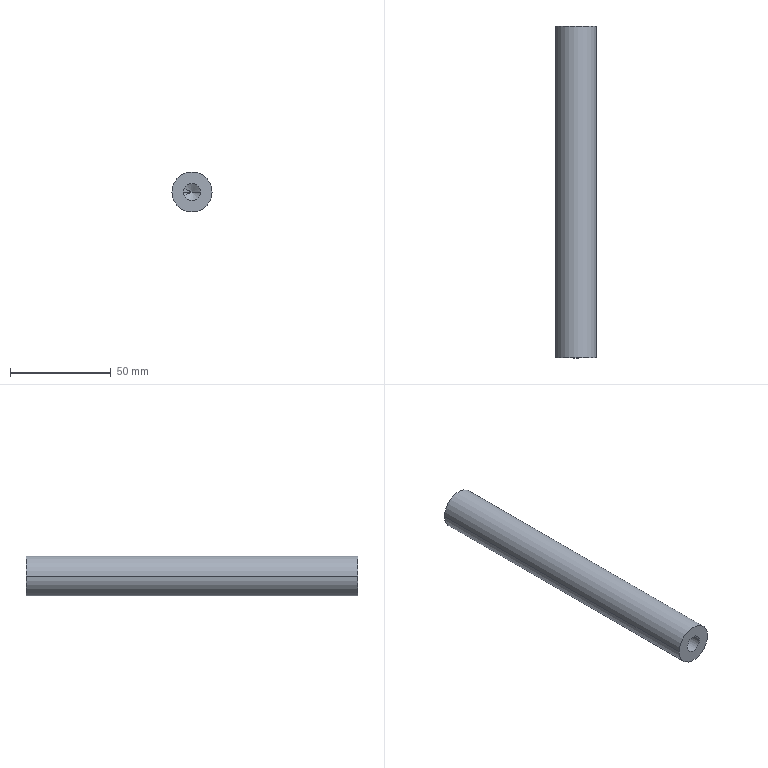Component | SolidWorks | YS01-055GuideRod2-1 | 1 solid | 12 faces | box 20 x 165 x 20 mm | volume 48959 mm3 | cylinder 6 | cone 4 | plane 2 | commonest cylinder face diameters 8.5 x4 20 x2
build123d program:
from build123d import *

# Parameters (mm, degrees)
SKETCH1_R              = 10
BOSS_EXTRUDE1_DEPTH    = 165
M10_TAPPED_HOLE1_D     = 8.5
M10_TAPPED_HOLE1_DEPTH = 24.5
M10_TAPPED_HOLE1_TIP   = 2.554
M10_TAPPED_HOLE2_D     = 8.5
M10_TAPPED_HOLE2_DEPTH = 24.5
M10_TAPPED_HOLE2_TIP   = 2.554


with BuildPart() as part:
    # Sketch1 → Boss-Extrude1 (new body)
    with BuildSketch(Plane.XY):
        with Locations((-44.896, -2.5)):
            Circle(SKETCH1_R)
    extrude(amount=BOSS_EXTRUDE1_DEPTH)

    # M10 Tapped Hole1
    with Locations(Plane(origin=(0, 0, 0), x_dir=(-1, 0, 0), z_dir=(0, 0, -1))):
        with Locations((44.896, -2.5)):
            Hole(M10_TAPPED_HOLE1_D / 2, depth=M10_TAPPED_HOLE1_DEPTH)
            with Locations((0, 0, -(M10_TAPPED_HOLE1_DEPTH + M10_TAPPED_HOLE1_TIP / 2))):  # 118° drill point
                Cone(0, M10_TAPPED_HOLE1_D / 2, M10_TAPPED_HOLE1_TIP, mode=Mode.SUBTRACT)

    # M10 Tapped Hole2
    with Locations(Plane.XY.offset(165)):
        with Locations((-44.896, -2.5)):
            Hole(M10_TAPPED_HOLE2_D / 2, depth=M10_TAPPED_HOLE2_DEPTH)
            with Locations((0, 0, -(M10_TAPPED_HOLE2_DEPTH + M10_TAPPED_HOLE2_TIP / 2))):  # 118° drill point
                Cone(0, M10_TAPPED_HOLE2_D / 2, M10_TAPPED_HOLE2_TIP, mode=Mode.SUBTRACT)


solid = part.part

# Placed as in the assembly
solid = solid.moved(Location((-596.716, -143.873, 2400.9), (90, 0, 0)))
STEP:
#1=COLOUR_RGB('',0.7922,0.8196,0.9333);
#2=FILL_AREA_STYLE_COLOUR('',#1);
#3=FILL_AREA_STYLE('',(#2));
#4=SURFACE_STYLE_FILL_AREA(#3);
#5=SURFACE_SIDE_STYLE('',(#4));
#6=SURFACE_STYLE_USAGE(.BOTH.,#5);
#7=PRESENTATION_STYLE_ASSIGNMENT((#6));
#8=CARTESIAN_POINT('',(-25.428,-6.629,94.425));
#9=VERTEX_POINT('',#8);
#10=CARTESIAN_POINT('',(-25.093,-6.629,94.425));
#11=VERTEX_POINT('',#10);
#12=CARTESIAN_POINT('',(-25.26,-6.629,94.425));
#13=DIRECTION('',(-0.,1.,0.));
#14=DIRECTION('',(1.,0.,0.));
#15=AXIS2_PLACEMENT_3D('',#12,#13,#14);
#16=CIRCLE('',#15,0.1673);
#17=EDGE_CURVE('',#9,#11,#16,.T.);
#18=ORIENTED_EDGE('',*,*,#17,.F.);
#19=CARTESIAN_POINT('',(-25.428,-5.664,94.425));
#20=VERTEX_POINT('',#19);
#21=CARTESIAN_POINT('',(-25.428,-5.664,94.425));
#22=DIRECTION('',(-0.,1.,0.));
#23=VECTOR('',#22,39.37);
#24=LINE('',#21,#23);
#25=EDGE_CURVE('',#9,#20,#24,.T.);
#26=ORIENTED_EDGE('',*,*,#25,.T.);
#27=CARTESIAN_POINT('',(-25.093,-5.664,94.425));
#28=VERTEX_POINT('',#27);
#29=CARTESIAN_POINT('',(-25.26,-5.664,94.425));
#30=DIRECTION('',(-0.,1.,0.));
#31=DIRECTION('',(1.,0.,0.));
#32=AXIS2_PLACEMENT_3D('',#29,#30,#31);
#33=CIRCLE('',#32,0.1673);
#34=EDGE_CURVE('',#20,#28,#33,.T.);
#35=ORIENTED_EDGE('',*,*,#34,.T.);
#36=CARTESIAN_POINT('',(-25.093,-5.664,94.425));
#37=DIRECTION('',(-0.,1.,0.));
#38=VECTOR('',#37,39.37);
#39=LINE('',#36,#38);
#40=EDGE_CURVE('',#11,#28,#39,.T.);
#41=ORIENTED_EDGE('',*,*,#40,.F.);
#42=EDGE_LOOP('',(#18,#26,#35,#41));
#43=FACE_OUTER_BOUND('',#42,.T.);
#44=CARTESIAN_POINT('',(-25.26,-5.664,94.425));
#45=DIRECTION('',(-0.,1.,0.));
#46=DIRECTION('',(1.,0.,0.));
#47=AXIS2_PLACEMENT_3D('',#44,#45,#46);
#48=CYLINDRICAL_SURFACE('',#47,0.1673);
#49=ADVANCED_FACE('',(#43),#48,.F.);
#50=CARTESIAN_POINT('',(-25.26,-6.729,94.425));
#51=VERTEX_POINT('',#50);
#52=CARTESIAN_POINT('',(-25.093,-6.629,94.425));
#53=DIRECTION('',(0.8572,0.515,0.));
#54=VECTOR('',#53,39.37);
#55=LINE('',#52,#54);
#56=EDGE_CURVE('',#51,#11,#55,.T.);
#57=ORIENTED_EDGE('',*,*,#56,.F.);
#58=CARTESIAN_POINT('',(-25.428,-6.629,94.425));
#59=DIRECTION('',(-0.8572,0.515,-0.));
#60=VECTOR('',#59,39.37);
#61=LINE('',#58,#60);
#62=EDGE_CURVE('',#51,#9,#61,.T.);
#63=ORIENTED_EDGE('',*,*,#62,.T.);
#64=ORIENTED_EDGE('',*,*,#17,.T.);
#65=EDGE_LOOP('',(#57,#63,#64));
#66=FACE_OUTER_BOUND('',#65,.T.);
#67=CARTESIAN_POINT('',(-25.26,-6.629,94.425));
#68=DIRECTION('',(-0.,1.,0.));
#69=DIRECTION('',(1.,0.,0.));
#70=AXIS2_PLACEMENT_3D('',#67,#68,#69);
#71=CONICAL_SURFACE('',#70,0.1673,1.03);
#72=ADVANCED_FACE('',(#66),#71,.F.);
#73=CARTESIAN_POINT('',(-25.093,-11.196,94.425));
#74=VERTEX_POINT('',#73);
#75=CARTESIAN_POINT('',(-25.428,-11.196,94.425));
#76=VERTEX_POINT('',#75);
#77=CARTESIAN_POINT('',(-25.26,-11.196,94.425));
#78=DIRECTION('',(0.,-1.,0.));
#79=DIRECTION('',(-1.,0.,0.));
#80=AXIS2_PLACEMENT_3D('',#77,#78,#79);
#81=CIRCLE('',#80,0.1673);
#82=EDGE_CURVE('',#74,#76,#81,.T.);
#83=ORIENTED_EDGE('',*,*,#82,.F.);
#84=CARTESIAN_POINT('',(-25.093,-12.16,94.425));
#85=VERTEX_POINT('',#84);
#86=CARTESIAN_POINT('',(-25.093,-12.16,94.425));
#87=DIRECTION('',(0.,-1.,0.));
#88=VECTOR('',#87,39.37);
#89=LINE('',#86,#88);
#90=EDGE_CURVE('',#74,#85,#89,.T.);
#91=ORIENTED_EDGE('',*,*,#90,.T.);
#92=CARTESIAN_POINT('',(-25.428,-12.16,94.425));
#93=VERTEX_POINT('',#92);
#94=CARTESIAN_POINT('',(-25.26,-12.16,94.425));
#95=DIRECTION('',(0.,-1.,0.));
#96=DIRECTION('',(-1.,0.,0.));
#97=AXIS2_PLACEMENT_3D('',#94,#95,#96);
#98=CIRCLE('',#97,0.1673);
#99=EDGE_CURVE('',#85,#93,#98,.T.);
#100=ORIENTED_EDGE('',*,*,#99,.T.);
#101=CARTESIAN_POINT('',(-25.428,-12.16,94.425));
#102=DIRECTION('',(0.,-1.,0.));
#103=VECTOR('',#102,39.37);
#104=LINE('',#101,#103);
#105=EDGE_CURVE('',#76,#93,#104,.T.);
#106=ORIENTED_EDGE('',*,*,#105,.F.);
#107=EDGE_LOOP('',(#83,#91,#100,#106));
#108=FACE_OUTER_BOUND('',#107,.T.);
#109=CARTESIAN_POINT('',(-25.26,-12.16,94.425));
#110=DIRECTION('',(0.,-1.,0.));
#111=DIRECTION('',(-1.,0.,0.));
#112=AXIS2_PLACEMENT_3D('',#109,#110,#111);
#113=CYLINDRICAL_SURFACE('',#112,0.1673);
#114=ADVANCED_FACE('',(#108),#113,.F.);
#115=CARTESIAN_POINT('',(-25.26,-11.095,94.425));
#116=VERTEX_POINT('',#115);
#117=CARTESIAN_POINT('',(-25.428,-11.196,94.425));
#118=DIRECTION('',(-0.8572,-0.515,0.));
#119=VECTOR('',#118,39.37);
#120=LINE('',#117,#119);
#121=EDGE_CURVE('',#116,#76,#120,.T.);
#122=ORIENTED_EDGE('',*,*,#121,.F.);
#123=CARTESIAN_POINT('',(-25.093,-11.196,94.425));
#124=DIRECTION('',(0.8572,-0.515,-0.));
#125=VECTOR('',#124,39.37);
#126=LINE('',#123,#125);
#127=EDGE_CURVE('',#116,#74,#126,.T.);
#128=ORIENTED_EDGE('',*,*,#127,.T.);
#129=ORIENTED_EDGE('',*,*,#82,.T.);
#130=EDGE_LOOP('',(#122,#128,#129));
#131=FACE_OUTER_BOUND('',#130,.T.);
#132=CARTESIAN_POINT('',(-25.26,-11.196,94.425));
#133=DIRECTION('',(0.,-1.,0.));
#134=DIRECTION('',(-1.,0.,0.));
#135=AXIS2_PLACEMENT_3D('',#132,#133,#134);
#136=CONICAL_SURFACE('',#135,0.1673,1.03);
#137=ADVANCED_FACE('',(#131),#136,.F.);
#138=CARTESIAN_POINT('',(-24.867,-5.664,94.425));
#139=VERTEX_POINT('',#138);
#140=CARTESIAN_POINT('',(-25.654,-5.664,94.425));
#141=VERTEX_POINT('',#140);
#142=CARTESIAN_POINT('',(-25.26,-5.664,94.425));
#143=DIRECTION('',(-0.,1.,0.));
#144=DIRECTION('',(1.,0.,0.));
#145=AXIS2_PLACEMENT_3D('',#142,#143,#144);
#146=CIRCLE('',#145,0.3937);
#147=EDGE_CURVE('',#139,#141,#146,.T.);
#148=ORIENTED_EDGE('',*,*,#147,.F.);
#149=CARTESIAN_POINT('',(-24.867,-12.16,94.425));
#150=VERTEX_POINT('',#149);
#151=CARTESIAN_POINT('',(-24.867,-5.664,94.425));
#152=DIRECTION('',(0.,-1.,0.));
#153=VECTOR('',#152,39.37);
#154=LINE('',#151,#153);
#155=EDGE_CURVE('',#139,#150,#154,.T.);
#156=ORIENTED_EDGE('',*,*,#155,.T.);
#157=CARTESIAN_POINT('',(-25.654,-12.16,94.425));
#158=VERTEX_POINT('',#157);
#159=CARTESIAN_POINT('',(-25.26,-12.16,94.425));
#160=DIRECTION('',(-0.,1.,0.));
#161=DIRECTION('',(1.,0.,0.));
#162=AXIS2_PLACEMENT_3D('',#159,#160,#161);
#163=CIRCLE('',#162,0.3937);
#164=EDGE_CURVE('',#150,#158,#163,.T.);
#165=ORIENTED_EDGE('',*,*,#164,.T.);
#166=CARTESIAN_POINT('',(-25.654,-5.664,94.425));
#167=DIRECTION('',(0.,-1.,0.));
#168=VECTOR('',#167,39.37);
#169=LINE('',#166,#168);
#170=EDGE_CURVE('',#141,#158,#169,.T.);
#171=ORIENTED_EDGE('',*,*,#170,.F.);
#172=EDGE_LOOP('',(#148,#156,#165,#171));
#173=FACE_OUTER_BOUND('',#172,.T.);
#174=CARTESIAN_POINT('',(-25.26,-5.664,94.425));
#175=DIRECTION('',(0.,-1.,0.));
#176=DIRECTION('',(-1.,0.,0.));
#177=AXIS2_PLACEMENT_3D('',#174,#175,#176);
#178=CYLINDRICAL_SURFACE('',#177,0.3937);
#179=ADVANCED_FACE('',(#173),#178,.T.);
#180=ORIENTED_EDGE('',*,*,#155,.F.);
#181=CARTESIAN_POINT('',(-25.26,-5.664,94.425));
#182=DIRECTION('',(-0.,1.,0.));
#183=DIRECTION('',(1.,0.,0.));
#184=AXIS2_PLACEMENT_3D('',#181,#182,#183);
#185=CIRCLE('',#184,0.3937);
#186=EDGE_CURVE('',#141,#139,#185,.T.);
#187=ORIENTED_EDGE('',*,*,#186,.F.);
#188=ORIENTED_EDGE('',*,*,#170,.T.);
#189=CARTESIAN_POINT('',(-25.26,-12.16,94.425));
#190=DIRECTION('',(-0.,1.,0.));
#191=DIRECTION('',(1.,0.,0.));
#192=AXIS2_PLACEMENT_3D('',#189,#190,#191);
#193=CIRCLE('',#192,0.3937);
#194=EDGE_CURVE('',#158,#150,#193,.T.);
#195=ORIENTED_EDGE('',*,*,#194,.T.);
#196=EDGE_LOOP('',(#180,#187,#188,#195));
#197=FACE_OUTER_BOUND('',#196,.T.);
#198=CARTESIAN_POINT('',(-25.26,-5.664,94.425));
#199=DIRECTION('',(0.,-1.,0.));
#200=DIRECTION('',(-1.,0.,0.));
#201=AXIS2_PLACEMENT_3D('',#198,#199,#200);
#202=CYLINDRICAL_SURFACE('',#201,0.3937);
#203=ADVANCED_FACE('',(#197),#202,.T.);
#204=CARTESIAN_POINT('',(-25.26,-5.664,94.425));
#205=DIRECTION('',(-0.,1.,0.));
#206=DIRECTION('',(1.,0.,0.));
#207=AXIS2_PLACEMENT_3D('',#204,#205,#206);
#208=CIRCLE('',#207,0.1673);
#209=EDGE_CURVE('',#28,#20,#208,.T.);
#210=ORIENTED_EDGE('',*,*,#209,.F.);
#211=ORIENTED_EDGE('',*,*,#34,.F.);
#212=EDGE_LOOP('',(#210,#211));
#213=FACE_BOUND('',#212,.T.);
#214=ORIENTED_EDGE('',*,*,#186,.T.);
#215=ORIENTED_EDGE('',*,*,#147,.T.);
#216=EDGE_LOOP('',(#214,#215));
#217=FACE_OUTER_BOUND('',#216,.T.);
#218=CARTESIAN_POINT('',(-25.26,-5.664,94.425));
#219=DIRECTION('',(-0.,1.,0.));
#220=DIRECTION('',(1.,0.,0.));
#221=AXIS2_PLACEMENT_3D('',#218,#219,#220);
#222=PLANE('',#221);
#223=ADVANCED_FACE('',(#213,#217),#222,.T.);
#224=CARTESIAN_POINT('',(-25.26,-12.16,94.425));
#225=DIRECTION('',(0.,-1.,0.));
#226=DIRECTION('',(-1.,0.,0.));
#227=AXIS2_PLACEMENT_3D('',#224,#225,#226);
#228=CIRCLE('',#227,0.1673);
#229=EDGE_CURVE('',#93,#85,#228,.T.);
#230=ORIENTED_EDGE('',*,*,#229,.F.);
#231=ORIENTED_EDGE('',*,*,#99,.F.);
#232=EDGE_LOOP('',(#230,#231));
#233=FACE_BOUND('',#232,.T.);
#234=ORIENTED_EDGE('',*,*,#194,.F.);
#235=ORIENTED_EDGE('',*,*,#164,.F.);
#236=EDGE_LOOP('',(#234,#235));
#237=FACE_OUTER_BOUND('',#236,.T.);
#238=CARTESIAN_POINT('',(-25.26,-12.16,94.425));
#239=DIRECTION('',(-0.,1.,0.));
#240=DIRECTION('',(1.,0.,0.));
#241=AXIS2_PLACEMENT_3D('',#238,#239,#240);
#242=PLANE('',#241);
#243=ADVANCED_FACE('',(#233,#237),#242,.F.);
#244=ORIENTED_EDGE('',*,*,#127,.F.);
#245=ORIENTED_EDGE('',*,*,#121,.T.);
#246=CARTESIAN_POINT('',(-25.26,-11.196,94.425));
#247=DIRECTION('',(0.,-1.,0.));
#248=DIRECTION('',(-1.,0.,0.));
#249=AXIS2_PLACEMENT_3D('',#246,#247,#248);
#250=CIRCLE('',#249,0.1673);
#251=EDGE_CURVE('',#76,#74,#250,.T.);
#252=ORIENTED_EDGE('',*,*,#251,.T.);
#253=EDGE_LOOP('',(#244,#245,#252));
#254=FACE_OUTER_BOUND('',#253,.T.);
#255=CARTESIAN_POINT('',(-25.26,-11.196,94.425));
#256=DIRECTION('',(0.,-1.,0.));
#257=DIRECTION('',(-1.,0.,0.));
#258=AXIS2_PLACEMENT_3D('',#255,#256,#257);
#259=CONICAL_SURFACE('',#258,0.1673,1.03);
#260=ADVANCED_FACE('',(#254),#259,.F.);
#261=ORIENTED_EDGE('',*,*,#90,.F.);
#262=ORIENTED_EDGE('',*,*,#251,.F.);
#263=ORIENTED_EDGE('',*,*,#105,.T.);
#264=ORIENTED_EDGE('',*,*,#229,.T.);
#265=EDGE_LOOP('',(#261,#262,#263,#264));
#266=FACE_OUTER_BOUND('',#265,.T.);
#267=CARTESIAN_POINT('',(-25.26,-12.16,94.425));
#268=DIRECTION('',(0.,-1.,0.));
#269=DIRECTION('',(-1.,0.,0.));
#270=AXIS2_PLACEMENT_3D('',#267,#268,#269);
#271=CYLINDRICAL_SURFACE('',#270,0.1673);
#272=ADVANCED_FACE('',(#266),#271,.F.);
#273=ORIENTED_EDGE('',*,*,#62,.F.);
#274=ORIENTED_EDGE('',*,*,#56,.T.);
#275=CARTESIAN_POINT('',(-25.26,-6.629,94.425));
#276=DIRECTION('',(-0.,1.,0.));
#277=DIRECTION('',(1.,0.,0.));
#278=AXIS2_PLACEMENT_3D('',#275,#276,#277);
#279=CIRCLE('',#278,0.1673);
#280=EDGE_CURVE('',#11,#9,#279,.T.);
#281=ORIENTED_EDGE('',*,*,#280,.T.);
#282=EDGE_LOOP('',(#273,#274,#281));
#283=FACE_OUTER_BOUND('',#282,.T.);
#284=CARTESIAN_POINT('',(-25.26,-6.629,94.425));
#285=DIRECTION('',(-0.,1.,0.));
#286=DIRECTION('',(1.,0.,0.));
#287=AXIS2_PLACEMENT_3D('',#284,#285,#286);
#288=CONICAL_SURFACE('',#287,0.1673,1.03);
#289=ADVANCED_FACE('',(#283),#288,.F.);
#290=ORIENTED_EDGE('',*,*,#25,.F.);
#291=ORIENTED_EDGE('',*,*,#280,.F.);
#292=ORIENTED_EDGE('',*,*,#40,.T.);
#293=ORIENTED_EDGE('',*,*,#209,.T.);
#294=EDGE_LOOP('',(#290,#291,#292,#293));
#295=FACE_OUTER_BOUND('',#294,.T.);
#296=CARTESIAN_POINT('',(-25.26,-5.664,94.425));
#297=DIRECTION('',(-0.,1.,0.));
#298=DIRECTION('',(1.,0.,0.));
#299=AXIS2_PLACEMENT_3D('',#296,#297,#298);
#300=CYLINDRICAL_SURFACE('',#299,0.1673);
#301=ADVANCED_FACE('',(#295),#300,.F.);
#302=CLOSED_SHELL('',(#49,#72,#114,#137,#179,#203,#223,#243,#260,#272,#289,#301));
#303=MANIFOLD_SOLID_BREP('',#302);
#304=STYLED_ITEM('',(#7),#303);
#305=(LENGTH_UNIT()NAMED_UNIT(*)SI_UNIT($,.METRE.));
#306=LENGTH_MEASURE_WITH_UNIT(LENGTH_MEASURE(0.0254),#305);
#307=DIMENSIONAL_EXPONENTS(1.,0.,0.,0.,0.,0.,0.);
#308=(CONVERSION_BASED_UNIT('',#306)LENGTH_UNIT()NAMED_UNIT(#307));
#309=UNCERTAINTY_MEASURE_WITH_UNIT(LENGTH_MEASURE(0.00001),#308,'','');
#310=(NAMED_UNIT(*)PLANE_ANGLE_UNIT()SI_UNIT($,.RADIAN.));
#311=(NAMED_UNIT(*)SI_UNIT($,.STERADIAN.)SOLID_ANGLE_UNIT());
#312=(GEOMETRIC_REPRESENTATION_CONTEXT(3)GLOBAL_UNCERTAINTY_ASSIGNED_CONTEXT((#309))GLOBAL_UNIT_ASSIGNED_CONTEXT((#308,#310,#311))REPRESENTATION_CONTEXT('',''));
#313=MECHANICAL_DESIGN_GEOMETRIC_PRESENTATION_REPRESENTATION('',(#304),#312);
#314=CARTESIAN_POINT('',(0.,0.,0.));
#315=DIRECTION('',(0.,0.,1.));
#316=DIRECTION('',(1.,0.,0.));
#317=AXIS2_PLACEMENT_3D('',#314,#315,#316);
#318=(LENGTH_UNIT()NAMED_UNIT(*)SI_UNIT($,.METRE.));
#319=LENGTH_MEASURE_WITH_UNIT(LENGTH_MEASURE(0.0254),#318);
#320=DIMENSIONAL_EXPONENTS(1.,0.,0.,0.,0.,0.,0.);
#321=(CONVERSION_BASED_UNIT('',#319)LENGTH_UNIT()NAMED_UNIT(#320));
#322=UNCERTAINTY_MEASURE_WITH_UNIT(LENGTH_MEASURE(0.00001),#321,'','');
#323=(NAMED_UNIT(*)PLANE_ANGLE_UNIT()SI_UNIT($,.RADIAN.));
#324=(NAMED_UNIT(*)SI_UNIT($,.STERADIAN.)SOLID_ANGLE_UNIT());
#325=(GEOMETRIC_REPRESENTATION_CONTEXT(3)GLOBAL_UNCERTAINTY_ASSIGNED_CONTEXT((#322))GLOBAL_UNIT_ASSIGNED_CONTEXT((#321,#323,#324))REPRESENTATION_CONTEXT('',''));
#326=ADVANCED_BREP_SHAPE_REPRESENTATION('',(#303,#317),#325);
#327=PRESENTATION_LAYER_ASSIGNMENT('','',(#304));